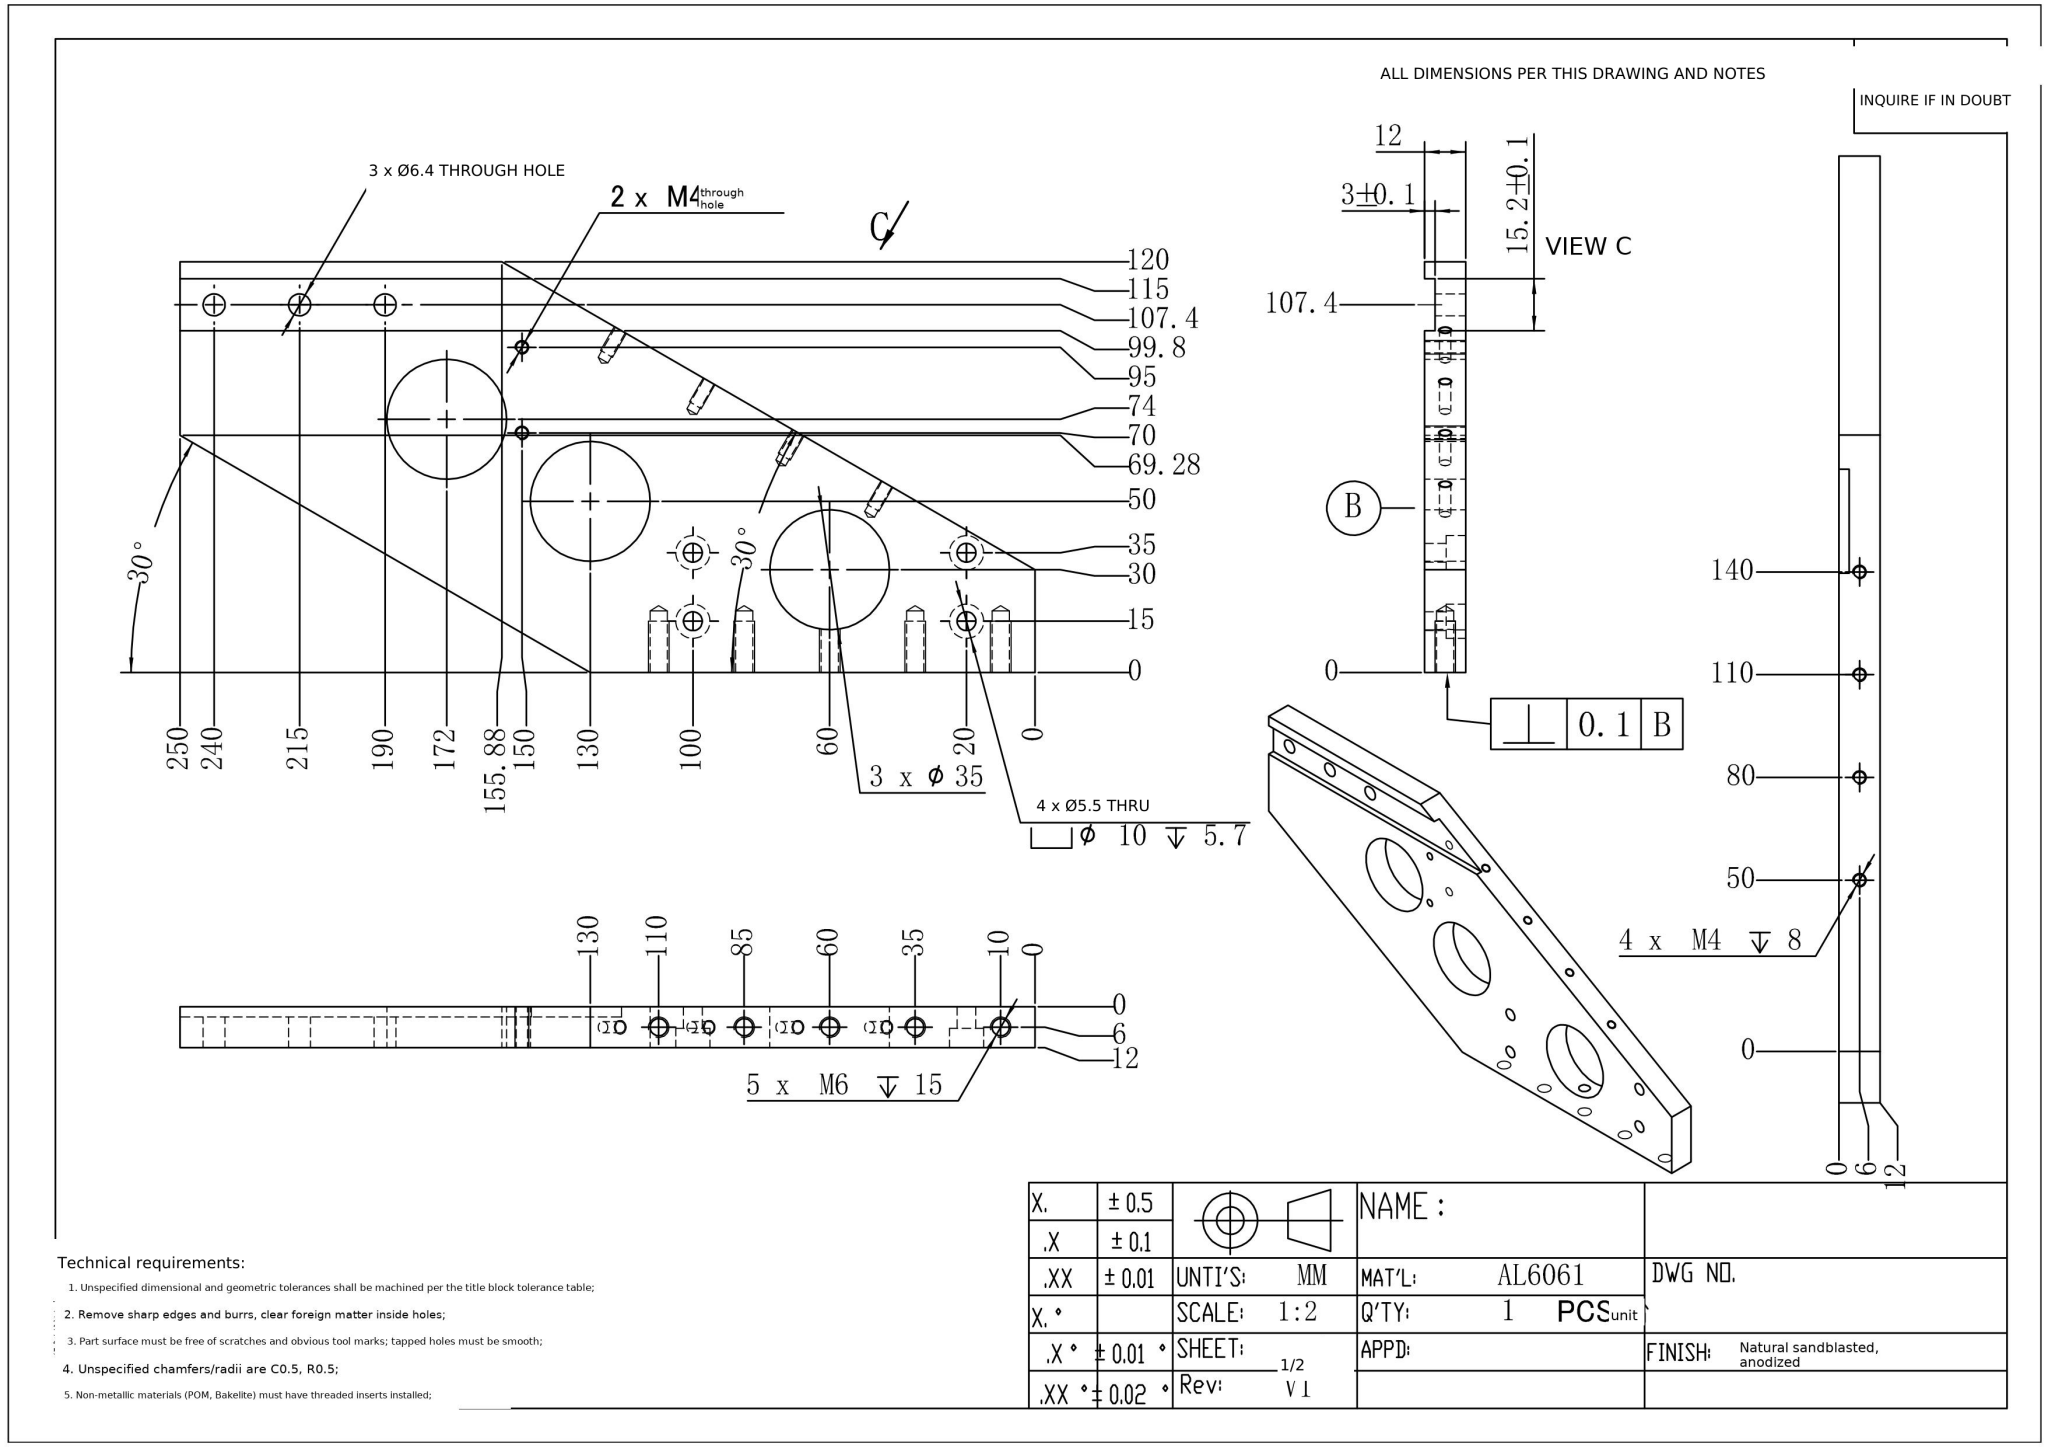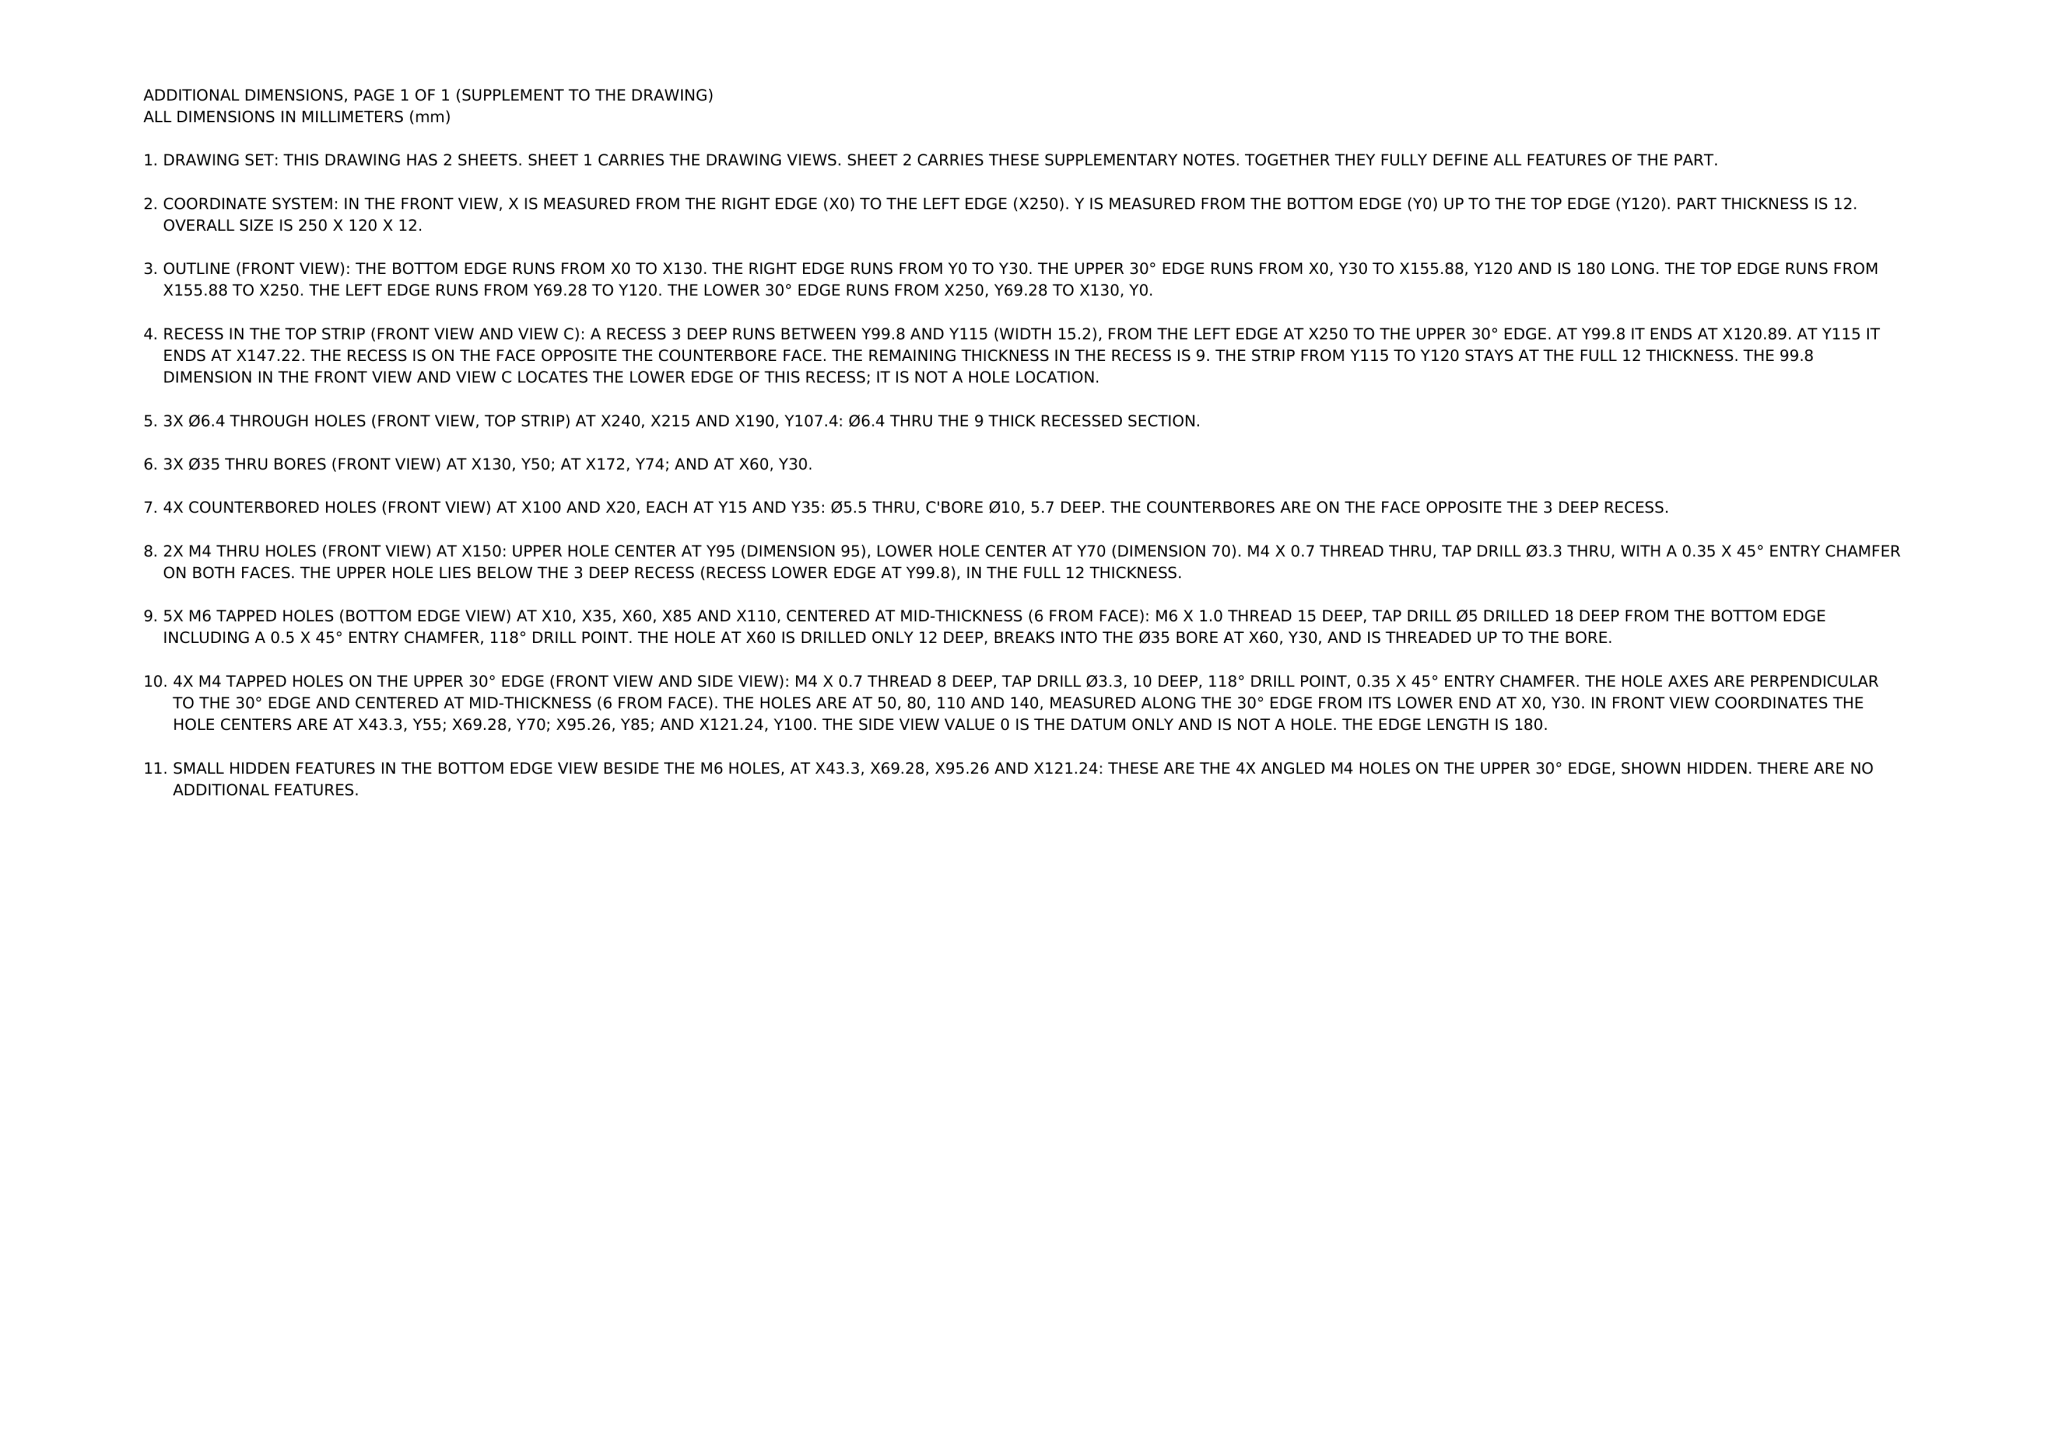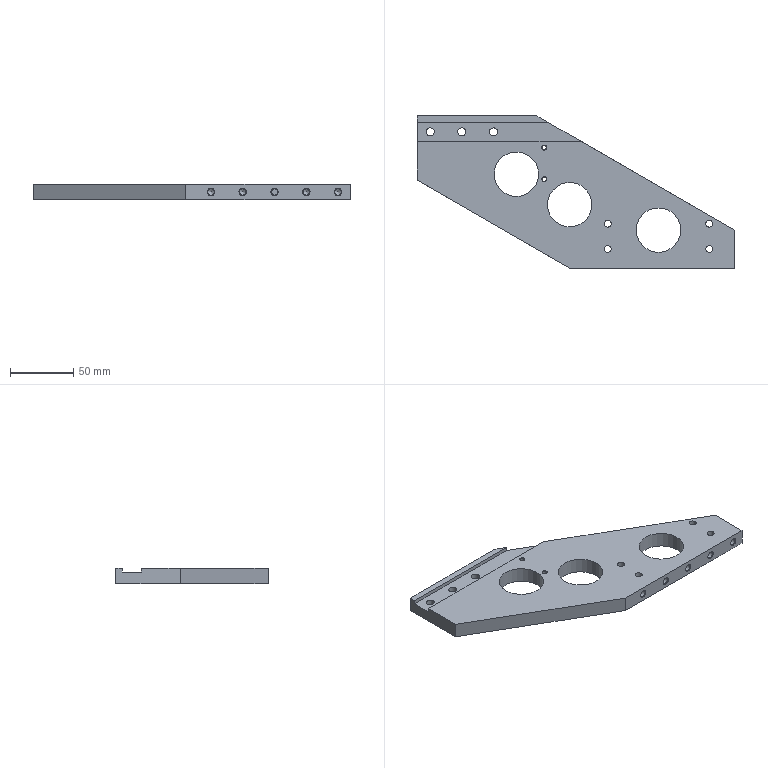Part | NX | mm | 1 solid | 63 faces | box 250 x 120 x 12 mm | volume 180485 mm3 | cylinder 25 | cone 22 | plane 16 | commonest cylinder face diameters 3.3 x6 5 x5 10 x4 5.5 x4 35 x3 6.4 x3